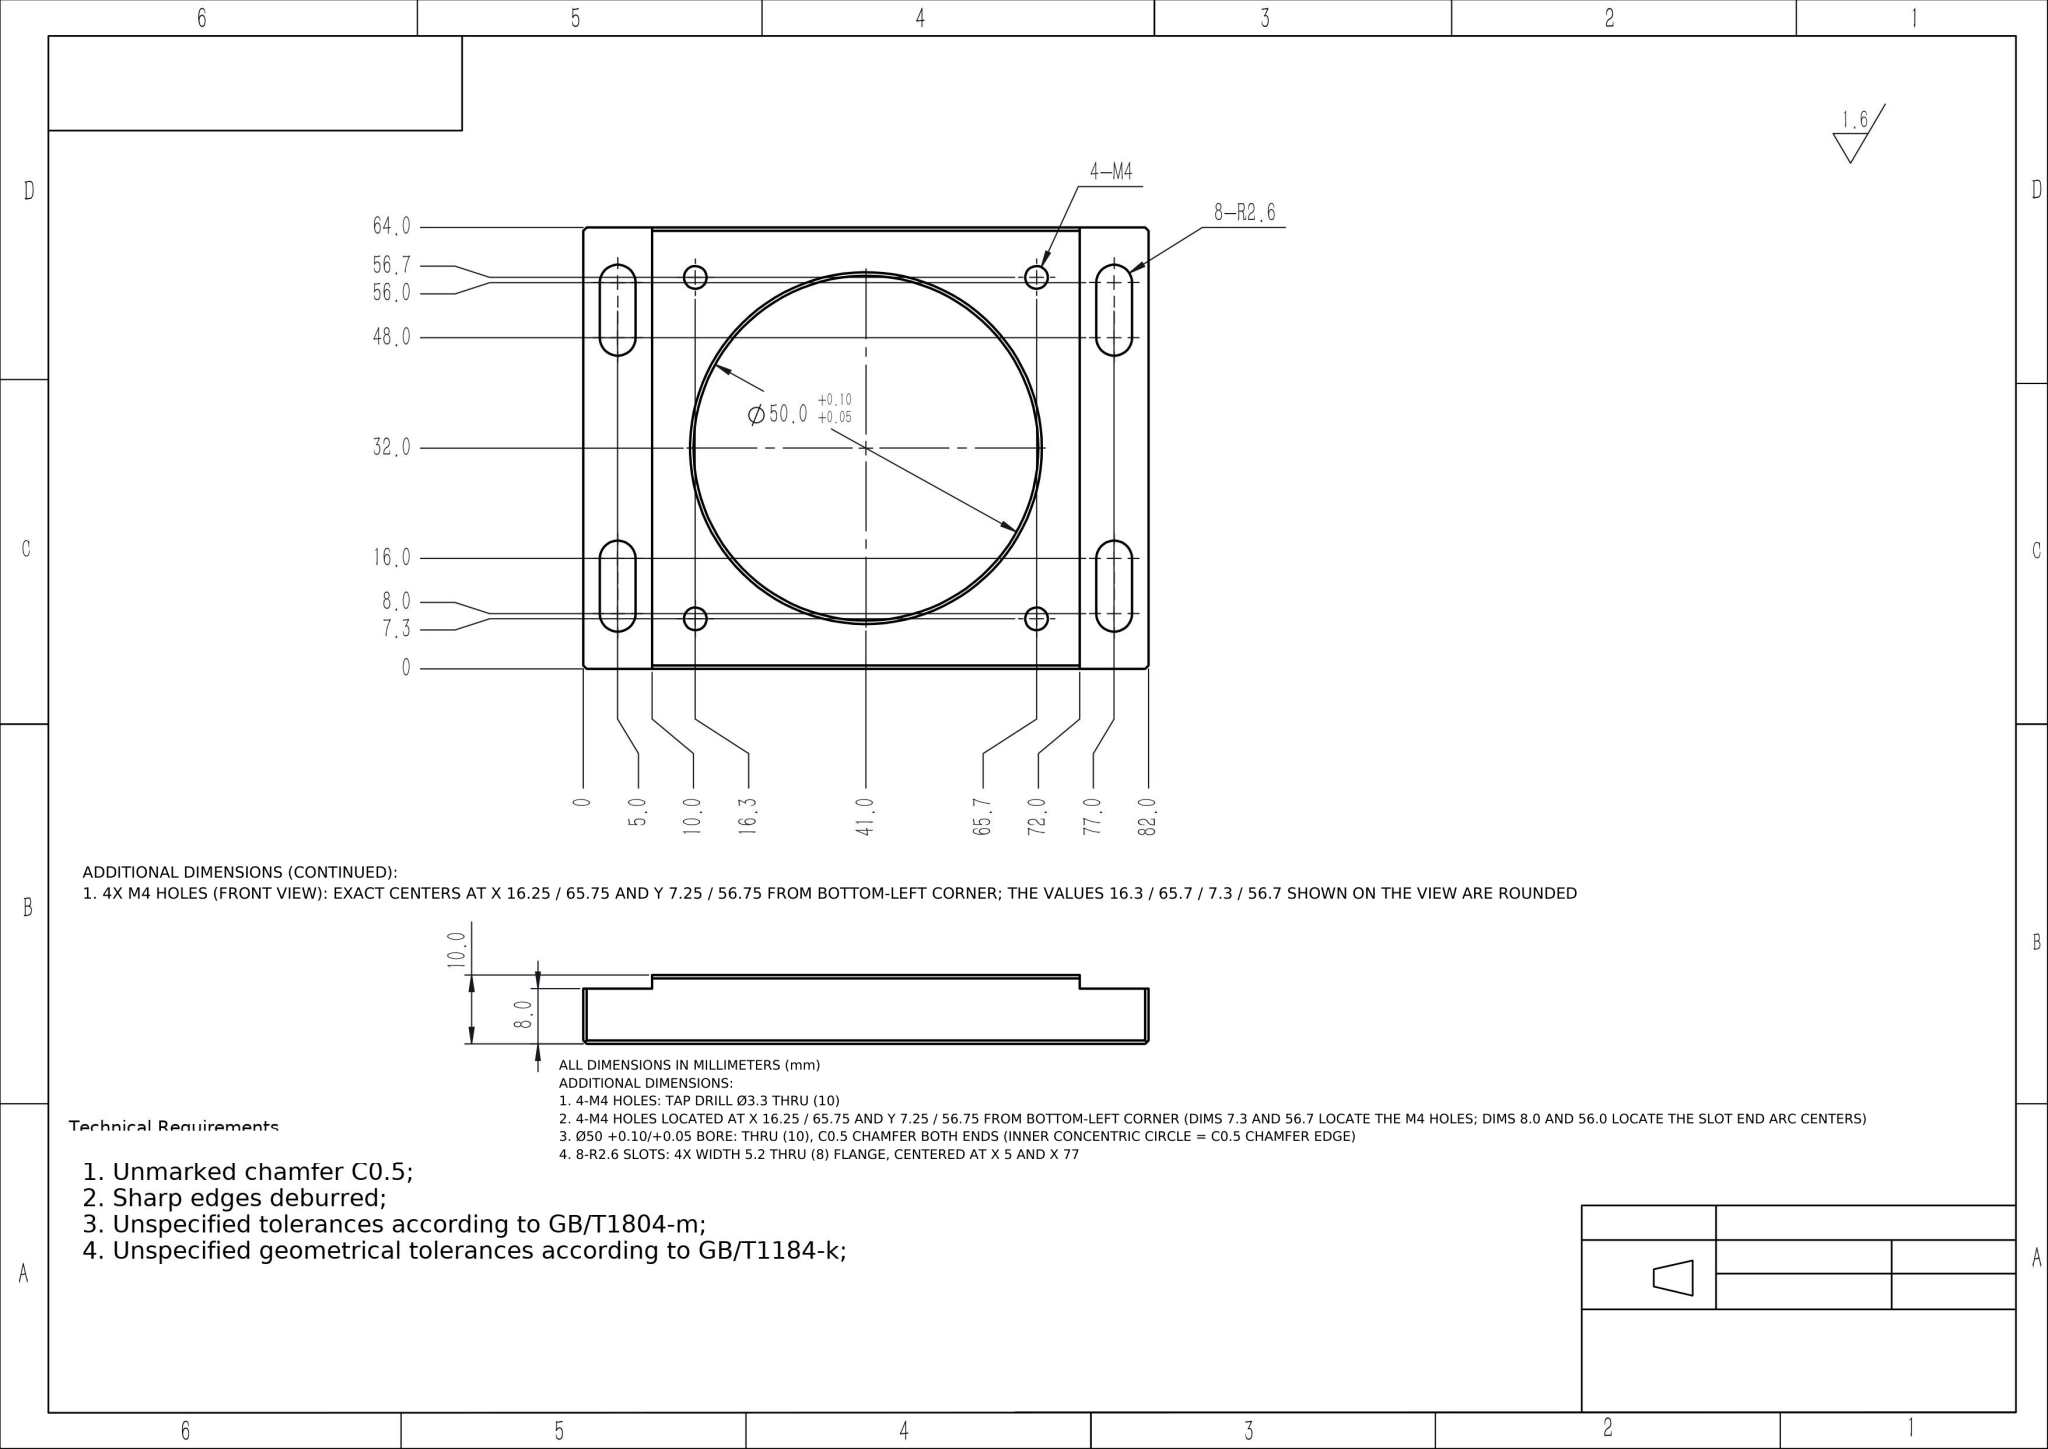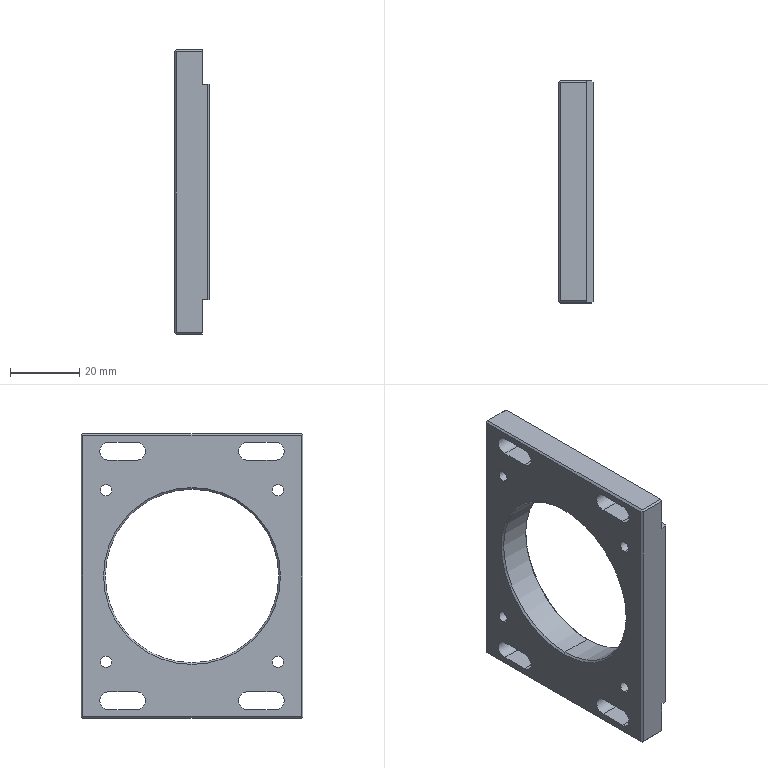Part | NX | mm | 1 solid | 50 faces | box 10 x 64 x 82 mm | volume 27837 mm3 | plane 28 | cylinder 18 | cone 4 | commonest cylinder face diameters 3.3 x8 5.2 x8 50 x2